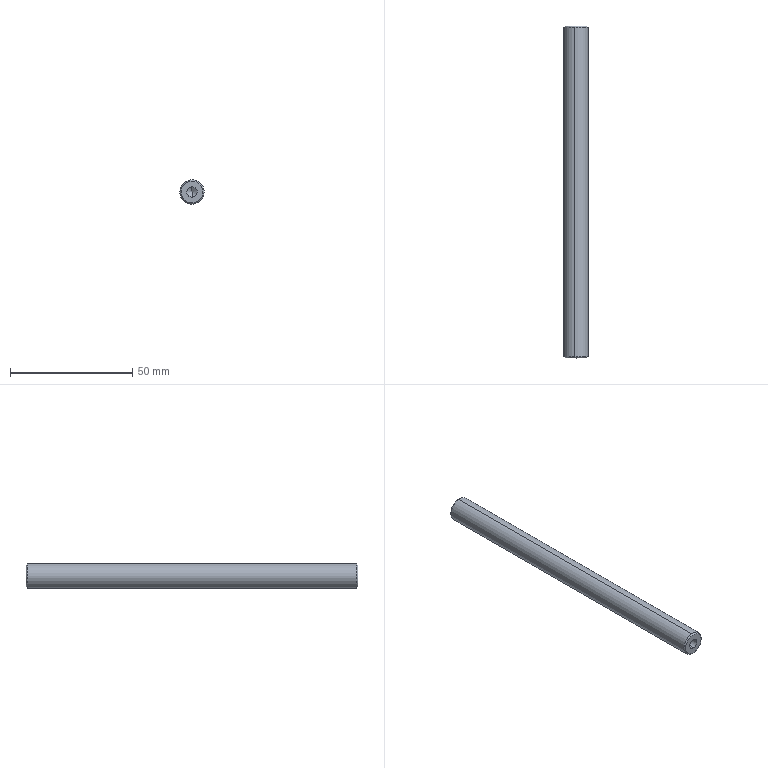Component | SolidWorks | BlankingGuidePost-136-1 | 1 solid | 16 faces | box 10 x 136 x 10 mm | volume 10319 mm3 | cone 8 | cylinder 6 | plane 2 | commonest cylinder face diameters 4.2 x4 10 x2 | material 45
build123d program:
from build123d import *

# Parameters (mm, degrees)
SKETCH1_R           = 5
BOSS_EXTRUDE1_DEPTH = 68
CHAMFER1_SIZE       = 0.5


with BuildPart() as part:
    # Sketch1 → Boss-Extrude1 (new, symmetric)
    with BuildSketch(Plane.XY):
        Circle(SKETCH1_R)
    extrude(amount=BOSS_EXTRUDE1_DEPTH, both=True)

    # Sketch4 → M5 Tapped Hole1 (revolve, cut)
    with BuildSketch(Plane(origin=(0, 0, 68), x_dir=(0, -1, 0), z_dir=(1, 0, 0))):
        Polygon((0, 0), (0, 13.662), (2.1, 12.4), (2.1, 0), align=None)
    m5_tapped_hole1 = revolve(axis=Axis((0, 0, 74.35), (0, 0, -1)), mode=Mode.SUBTRACT)

    # Mirror1: M5 Tapped Hole1 across plane
    add(m5_tapped_hole1.mirror(Plane.XY), mode=Mode.SUBTRACT)

    # Chamfer1
    chamfer1_edges = [part.edges().sort_by_distance(p)[0] for p in [
        (-5, 0, -68),
        (-5, 0, 68),
    ]]
    chamfer(chamfer1_edges, length=CHAMFER1_SIZE)


solid = part.part

# Placed as in the assembly
solid = solid.moved(Location((0, -25, -30), (90, 0, 0)))
STEP:
#1=CARTESIAN_POINT('',(-0.01499,-3.661,-1.005));
#2=VERTEX_POINT('',#1);
#3=CARTESIAN_POINT('',(0.01499,-3.661,-1.358));
#4=VERTEX_POINT('',#3);
#5=CARTESIAN_POINT('',(-0.,-3.661,-1.181));
#6=DIRECTION('',(0.,-1.,-0.));
#7=DIRECTION('',(-0.08459,0.,0.9964));
#8=AXIS2_PLACEMENT_3D('',#5,#6,#7);
#9=CIRCLE('',#8,0.1772);
#10=EDGE_CURVE('',#2,#4,#9,.T.);
#11=ORIENTED_EDGE('',*,*,#10,.F.);
#12=CARTESIAN_POINT('',(-0.01665,-3.642,-0.985));
#13=VERTEX_POINT('',#12);
#14=CARTESIAN_POINT('',(-0.01499,-3.661,-1.005));
#15=DIRECTION('',(-0.05981,0.7071,0.7046));
#16=VECTOR('',#15,39.37);
#17=LINE('',#14,#16);
#18=EDGE_CURVE('',#2,#13,#17,.T.);
#19=ORIENTED_EDGE('',*,*,#18,.T.);
#20=CARTESIAN_POINT('',(0.01665,-3.642,-1.377));
#21=VERTEX_POINT('',#20);
#22=CARTESIAN_POINT('',(-0.,-3.642,-1.181));
#23=DIRECTION('',(-0.,1.,0.));
#24=DIRECTION('',(-0.08459,0.,0.9964));
#25=AXIS2_PLACEMENT_3D('',#22,#23,#24);
#26=CIRCLE('',#25,0.1969);
#27=EDGE_CURVE('',#21,#13,#26,.T.);
#28=ORIENTED_EDGE('',*,*,#27,.F.);
#29=CARTESIAN_POINT('',(0.01499,-3.661,-1.358));
#30=DIRECTION('',(0.05981,0.7071,-0.7046));
#31=VECTOR('',#30,39.37);
#32=LINE('',#29,#31);
#33=EDGE_CURVE('',#4,#21,#32,.T.);
#34=ORIENTED_EDGE('',*,*,#33,.F.);
#35=EDGE_LOOP('',(#11,#19,#28,#34));
#36=FACE_OUTER_BOUND('',#35,.T.);
#37=CARTESIAN_POINT('',(-0.,-3.661,-1.181));
#38=DIRECTION('',(-0.,1.,0.));
#39=DIRECTION('',(0.08459,0.,-0.9964));
#40=AXIS2_PLACEMENT_3D('',#37,#38,#39);
#41=CONICAL_SURFACE('',#40,0.1772,0.7854);
#42=ADVANCED_FACE('',(#36),#41,.T.);
#43=CARTESIAN_POINT('',(0.01499,1.693,-1.358));
#44=VERTEX_POINT('',#43);
#45=CARTESIAN_POINT('',(-0.01499,1.693,-1.005));
#46=VERTEX_POINT('',#45);
#47=CARTESIAN_POINT('',(-0.,1.693,-1.181));
#48=DIRECTION('',(-0.,1.,0.));
#49=DIRECTION('',(-0.08459,0.,0.9964));
#50=AXIS2_PLACEMENT_3D('',#47,#48,#49);
#51=CIRCLE('',#50,0.1772);
#52=EDGE_CURVE('',#44,#46,#51,.T.);
#53=ORIENTED_EDGE('',*,*,#52,.F.);
#54=CARTESIAN_POINT('',(0.01665,1.673,-1.377));
#55=VERTEX_POINT('',#54);
#56=CARTESIAN_POINT('',(0.01665,1.673,-1.377));
#57=DIRECTION('',(0.05981,-0.7071,-0.7046));
#58=VECTOR('',#57,39.37);
#59=LINE('',#56,#58);
#60=EDGE_CURVE('',#44,#55,#59,.T.);
#61=ORIENTED_EDGE('',*,*,#60,.T.);
#62=CARTESIAN_POINT('',(-0.01665,1.673,-0.985));
#63=VERTEX_POINT('',#62);
#64=CARTESIAN_POINT('',(-0.,1.673,-1.181));
#65=DIRECTION('',(0.,-1.,-0.));
#66=DIRECTION('',(-0.08459,0.,0.9964));
#67=AXIS2_PLACEMENT_3D('',#64,#65,#66);
#68=CIRCLE('',#67,0.1969);
#69=EDGE_CURVE('',#63,#55,#68,.T.);
#70=ORIENTED_EDGE('',*,*,#69,.F.);
#71=CARTESIAN_POINT('',(-0.01665,1.673,-0.985));
#72=DIRECTION('',(-0.05981,-0.7071,0.7046));
#73=VECTOR('',#72,39.37);
#74=LINE('',#71,#73);
#75=EDGE_CURVE('',#46,#63,#74,.T.);
#76=ORIENTED_EDGE('',*,*,#75,.F.);
#77=EDGE_LOOP('',(#53,#61,#70,#76));
#78=FACE_OUTER_BOUND('',#77,.T.);
#79=CARTESIAN_POINT('',(-0.,1.673,-1.181));
#80=DIRECTION('',(0.,-1.,-0.));
#81=DIRECTION('',(-0.08459,0.,0.9964));
#82=AXIS2_PLACEMENT_3D('',#79,#80,#81);
#83=CONICAL_SURFACE('',#82,0.1969,0.7854);
#84=ADVANCED_FACE('',(#78),#83,.T.);
#85=CARTESIAN_POINT('',(-0.006994,1.205,-1.099));
#86=VERTEX_POINT('',#85);
#87=CARTESIAN_POINT('',(0.006994,1.205,-1.263));
#88=VERTEX_POINT('',#87);
#89=CARTESIAN_POINT('',(-0.,1.205,-1.181));
#90=DIRECTION('',(-0.,1.,0.));
#91=DIRECTION('',(0.08459,0.,-0.9964));
#92=AXIS2_PLACEMENT_3D('',#89,#90,#91);
#93=CIRCLE('',#92,0.08268);
#94=EDGE_CURVE('',#86,#88,#93,.T.);
#95=ORIENTED_EDGE('',*,*,#94,.F.);
#96=CARTESIAN_POINT('',(-0.006994,1.693,-1.099));
#97=VERTEX_POINT('',#96);
#98=CARTESIAN_POINT('',(-0.006994,1.693,-1.099));
#99=DIRECTION('',(-0.,1.,0.));
#100=VECTOR('',#99,39.37);
#101=LINE('',#98,#100);
#102=EDGE_CURVE('',#86,#97,#101,.T.);
#103=ORIENTED_EDGE('',*,*,#102,.T.);
#104=CARTESIAN_POINT('',(0.006994,1.693,-1.263));
#105=VERTEX_POINT('',#104);
#106=CARTESIAN_POINT('',(-0.,1.693,-1.181));
#107=DIRECTION('',(-0.,1.,0.));
#108=DIRECTION('',(0.08459,0.,-0.9964));
#109=AXIS2_PLACEMENT_3D('',#106,#107,#108);
#110=CIRCLE('',#109,0.08268);
#111=EDGE_CURVE('',#97,#105,#110,.T.);
#112=ORIENTED_EDGE('',*,*,#111,.T.);
#113=CARTESIAN_POINT('',(0.006994,1.693,-1.263));
#114=DIRECTION('',(-0.,1.,0.));
#115=VECTOR('',#114,39.37);
#116=LINE('',#113,#115);
#117=EDGE_CURVE('',#88,#105,#116,.T.);
#118=ORIENTED_EDGE('',*,*,#117,.F.);
#119=EDGE_LOOP('',(#95,#103,#112,#118));
#120=FACE_OUTER_BOUND('',#119,.T.);
#121=CARTESIAN_POINT('',(-0.,1.693,-1.181));
#122=DIRECTION('',(-0.,1.,0.));
#123=DIRECTION('',(0.08459,0.,-0.9964));
#124=AXIS2_PLACEMENT_3D('',#121,#122,#123);
#125=CYLINDRICAL_SURFACE('',#124,0.08268);
#126=ADVANCED_FACE('',(#120),#125,.F.);
#127=CARTESIAN_POINT('',(-0.,1.155,-1.181));
#128=VERTEX_POINT('',#127);
#129=CARTESIAN_POINT('',(0.006994,1.205,-1.263));
#130=DIRECTION('',(0.07251,0.515,-0.8541));
#131=VECTOR('',#130,39.37);
#132=LINE('',#129,#131);
#133=EDGE_CURVE('',#128,#88,#132,.T.);
#134=ORIENTED_EDGE('',*,*,#133,.F.);
#135=CARTESIAN_POINT('',(-0.006994,1.205,-1.099));
#136=DIRECTION('',(-0.07251,0.515,0.8541));
#137=VECTOR('',#136,39.37);
#138=LINE('',#135,#137);
#139=EDGE_CURVE('',#128,#86,#138,.T.);
#140=ORIENTED_EDGE('',*,*,#139,.T.);
#141=ORIENTED_EDGE('',*,*,#94,.T.);
#142=EDGE_LOOP('',(#134,#140,#141));
#143=FACE_OUTER_BOUND('',#142,.T.);
#144=CARTESIAN_POINT('',(-0.,1.205,-1.181));
#145=DIRECTION('',(-0.,1.,0.));
#146=DIRECTION('',(0.08459,0.,-0.9964));
#147=AXIS2_PLACEMENT_3D('',#144,#145,#146);
#148=CONICAL_SURFACE('',#147,0.08268,1.03);
#149=ADVANCED_FACE('',(#143),#148,.F.);
#150=CARTESIAN_POINT('',(0.006994,-3.173,-1.263));
#151=VERTEX_POINT('',#150);
#152=CARTESIAN_POINT('',(-0.006994,-3.173,-1.099));
#153=VERTEX_POINT('',#152);
#154=CARTESIAN_POINT('',(-0.,-3.173,-1.181));
#155=DIRECTION('',(0.,-1.,-0.));
#156=DIRECTION('',(-0.08459,0.,0.9964));
#157=AXIS2_PLACEMENT_3D('',#154,#155,#156);
#158=CIRCLE('',#157,0.08268);
#159=EDGE_CURVE('',#151,#153,#158,.T.);
#160=ORIENTED_EDGE('',*,*,#159,.F.);
#161=CARTESIAN_POINT('',(0.006994,-3.661,-1.263));
#162=VERTEX_POINT('',#161);
#163=CARTESIAN_POINT('',(0.006994,-3.661,-1.263));
#164=DIRECTION('',(0.,-1.,-0.));
#165=VECTOR('',#164,39.37);
#166=LINE('',#163,#165);
#167=EDGE_CURVE('',#151,#162,#166,.T.);
#168=ORIENTED_EDGE('',*,*,#167,.T.);
#169=CARTESIAN_POINT('',(-0.006994,-3.661,-1.099));
#170=VERTEX_POINT('',#169);
#171=CARTESIAN_POINT('',(-0.,-3.661,-1.181));
#172=DIRECTION('',(0.,-1.,-0.));
#173=DIRECTION('',(-0.08459,0.,0.9964));
#174=AXIS2_PLACEMENT_3D('',#171,#172,#173);
#175=CIRCLE('',#174,0.08268);
#176=EDGE_CURVE('',#162,#170,#175,.T.);
#177=ORIENTED_EDGE('',*,*,#176,.T.);
#178=CARTESIAN_POINT('',(-0.006994,-3.661,-1.099));
#179=DIRECTION('',(0.,-1.,-0.));
#180=VECTOR('',#179,39.37);
#181=LINE('',#178,#180);
#182=EDGE_CURVE('',#153,#170,#181,.T.);
#183=ORIENTED_EDGE('',*,*,#182,.F.);
#184=EDGE_LOOP('',(#160,#168,#177,#183));
#185=FACE_OUTER_BOUND('',#184,.T.);
#186=CARTESIAN_POINT('',(-0.,-3.661,-1.181));
#187=DIRECTION('',(0.,-1.,-0.));
#188=DIRECTION('',(-0.08459,0.,0.9964));
#189=AXIS2_PLACEMENT_3D('',#186,#187,#188);
#190=CYLINDRICAL_SURFACE('',#189,0.08268);
#191=ADVANCED_FACE('',(#185),#190,.F.);
#192=CARTESIAN_POINT('',(-0.,-3.124,-1.181));
#193=VERTEX_POINT('',#192);
#194=CARTESIAN_POINT('',(-0.006994,-3.173,-1.099));
#195=DIRECTION('',(-0.07251,-0.515,0.8541));
#196=VECTOR('',#195,39.37);
#197=LINE('',#194,#196);
#198=EDGE_CURVE('',#193,#153,#197,.T.);
#199=ORIENTED_EDGE('',*,*,#198,.F.);
#200=CARTESIAN_POINT('',(0.006994,-3.173,-1.263));
#201=DIRECTION('',(0.07251,-0.515,-0.8541));
#202=VECTOR('',#201,39.37);
#203=LINE('',#200,#202);
#204=EDGE_CURVE('',#193,#151,#203,.T.);
#205=ORIENTED_EDGE('',*,*,#204,.T.);
#206=ORIENTED_EDGE('',*,*,#159,.T.);
#207=EDGE_LOOP('',(#199,#205,#206));
#208=FACE_OUTER_BOUND('',#207,.T.);
#209=CARTESIAN_POINT('',(-0.,-3.173,-1.181));
#210=DIRECTION('',(0.,-1.,-0.));
#211=DIRECTION('',(-0.08459,0.,0.9964));
#212=AXIS2_PLACEMENT_3D('',#209,#210,#211);
#213=CONICAL_SURFACE('',#212,0.08268,1.03);
#214=ADVANCED_FACE('',(#208),#213,.F.);
#215=ORIENTED_EDGE('',*,*,#27,.T.);
#216=CARTESIAN_POINT('',(-0.01665,-3.661,-0.985));
#217=DIRECTION('',(-0.,1.,0.));
#218=VECTOR('',#217,39.37);
#219=LINE('',#216,#218);
#220=EDGE_CURVE('',#13,#63,#219,.T.);
#221=ORIENTED_EDGE('',*,*,#220,.T.);
#222=ORIENTED_EDGE('',*,*,#69,.T.);
#223=CARTESIAN_POINT('',(0.01665,-3.661,-1.377));
#224=DIRECTION('',(-0.,1.,0.));
#225=VECTOR('',#224,39.37);
#226=LINE('',#223,#225);
#227=EDGE_CURVE('',#21,#55,#226,.T.);
#228=ORIENTED_EDGE('',*,*,#227,.F.);
#229=EDGE_LOOP('',(#215,#221,#222,#228));
#230=FACE_OUTER_BOUND('',#229,.T.);
#231=CARTESIAN_POINT('',(-0.,-3.661,-1.181));
#232=DIRECTION('',(-0.,1.,0.));
#233=DIRECTION('',(0.08459,0.,-0.9964));
#234=AXIS2_PLACEMENT_3D('',#231,#232,#233);
#235=CYLINDRICAL_SURFACE('',#234,0.1969);
#236=ADVANCED_FACE('',(#230),#235,.T.);
#237=ORIENTED_EDGE('',*,*,#220,.F.);
#238=CARTESIAN_POINT('',(-0.,-3.642,-1.181));
#239=DIRECTION('',(-0.,1.,0.));
#240=DIRECTION('',(-0.08459,0.,0.9964));
#241=AXIS2_PLACEMENT_3D('',#238,#239,#240);
#242=CIRCLE('',#241,0.1969);
#243=EDGE_CURVE('',#13,#21,#242,.T.);
#244=ORIENTED_EDGE('',*,*,#243,.T.);
#245=ORIENTED_EDGE('',*,*,#227,.T.);
#246=CARTESIAN_POINT('',(-0.,1.673,-1.181));
#247=DIRECTION('',(0.,-1.,-0.));
#248=DIRECTION('',(-0.08459,0.,0.9964));
#249=AXIS2_PLACEMENT_3D('',#246,#247,#248);
#250=CIRCLE('',#249,0.1969);
#251=EDGE_CURVE('',#55,#63,#250,.T.);
#252=ORIENTED_EDGE('',*,*,#251,.T.);
#253=EDGE_LOOP('',(#237,#244,#245,#252));
#254=FACE_OUTER_BOUND('',#253,.T.);
#255=CARTESIAN_POINT('',(-0.,-3.661,-1.181));
#256=DIRECTION('',(-0.,1.,0.));
#257=DIRECTION('',(0.08459,0.,-0.9964));
#258=AXIS2_PLACEMENT_3D('',#255,#256,#257);
#259=CYLINDRICAL_SURFACE('',#258,0.1969);
#260=ADVANCED_FACE('',(#254),#259,.T.);
#261=CARTESIAN_POINT('',(-0.,-3.661,-1.181));
#262=DIRECTION('',(0.,-1.,-0.));
#263=DIRECTION('',(-0.08459,0.,0.9964));
#264=AXIS2_PLACEMENT_3D('',#261,#262,#263);
#265=CIRCLE('',#264,0.1772);
#266=EDGE_CURVE('',#4,#2,#265,.T.);
#267=ORIENTED_EDGE('',*,*,#266,.T.);
#268=ORIENTED_EDGE('',*,*,#10,.T.);
#269=EDGE_LOOP('',(#267,#268));
#270=FACE_OUTER_BOUND('',#269,.T.);
#271=CARTESIAN_POINT('',(-0.,-3.661,-1.181));
#272=DIRECTION('',(0.,-1.,-0.));
#273=DIRECTION('',(-0.08459,0.,0.9964));
#274=AXIS2_PLACEMENT_3D('',#271,#272,#273);
#275=CIRCLE('',#274,0.08268);
#276=EDGE_CURVE('',#170,#162,#275,.T.);
#277=ORIENTED_EDGE('',*,*,#276,.F.);
#278=ORIENTED_EDGE('',*,*,#176,.F.);
#279=EDGE_LOOP('',(#277,#278));
#280=FACE_BOUND('',#279,.T.);
#281=CARTESIAN_POINT('',(-0.,-3.661,-1.181));
#282=DIRECTION('',(0.,-1.,-0.));
#283=DIRECTION('',(-0.08459,-0.,0.9964));
#284=AXIS2_PLACEMENT_3D('',#281,#282,#283);
#285=PLANE('',#284);
#286=ADVANCED_FACE('',(#270,#280),#285,.T.);
#287=CARTESIAN_POINT('',(-0.,1.693,-1.181));
#288=DIRECTION('',(-0.,1.,0.));
#289=DIRECTION('',(-0.08459,0.,0.9964));
#290=AXIS2_PLACEMENT_3D('',#287,#288,#289);
#291=CIRCLE('',#290,0.1772);
#292=EDGE_CURVE('',#46,#44,#291,.T.);
#293=ORIENTED_EDGE('',*,*,#292,.T.);
#294=ORIENTED_EDGE('',*,*,#52,.T.);
#295=EDGE_LOOP('',(#293,#294));
#296=FACE_OUTER_BOUND('',#295,.T.);
#297=CARTESIAN_POINT('',(-0.,1.693,-1.181));
#298=DIRECTION('',(-0.,1.,0.));
#299=DIRECTION('',(0.08459,0.,-0.9964));
#300=AXIS2_PLACEMENT_3D('',#297,#298,#299);
#301=CIRCLE('',#300,0.08268);
#302=EDGE_CURVE('',#105,#97,#301,.T.);
#303=ORIENTED_EDGE('',*,*,#302,.F.);
#304=ORIENTED_EDGE('',*,*,#111,.F.);
#305=EDGE_LOOP('',(#303,#304));
#306=FACE_BOUND('',#305,.T.);
#307=CARTESIAN_POINT('',(-0.,1.693,-1.181));
#308=DIRECTION('',(0.,-1.,-0.));
#309=DIRECTION('',(-0.08459,-0.,0.9964));
#310=AXIS2_PLACEMENT_3D('',#307,#308,#309);
#311=PLANE('',#310);
#312=ADVANCED_FACE('',(#296,#306),#311,.F.);
#313=ORIENTED_EDGE('',*,*,#204,.F.);
#314=ORIENTED_EDGE('',*,*,#198,.T.);
#315=CARTESIAN_POINT('',(-0.,-3.173,-1.181));
#316=DIRECTION('',(0.,-1.,-0.));
#317=DIRECTION('',(-0.08459,0.,0.9964));
#318=AXIS2_PLACEMENT_3D('',#315,#316,#317);
#319=CIRCLE('',#318,0.08268);
#320=EDGE_CURVE('',#153,#151,#319,.T.);
#321=ORIENTED_EDGE('',*,*,#320,.T.);
#322=EDGE_LOOP('',(#313,#314,#321));
#323=FACE_OUTER_BOUND('',#322,.T.);
#324=CARTESIAN_POINT('',(-0.,-3.173,-1.181));
#325=DIRECTION('',(0.,-1.,-0.));
#326=DIRECTION('',(-0.08459,0.,0.9964));
#327=AXIS2_PLACEMENT_3D('',#324,#325,#326);
#328=CONICAL_SURFACE('',#327,0.08268,1.03);
#329=ADVANCED_FACE('',(#323),#328,.F.);
#330=ORIENTED_EDGE('',*,*,#167,.F.);
#331=ORIENTED_EDGE('',*,*,#320,.F.);
#332=ORIENTED_EDGE('',*,*,#182,.T.);
#333=ORIENTED_EDGE('',*,*,#276,.T.);
#334=EDGE_LOOP('',(#330,#331,#332,#333));
#335=FACE_OUTER_BOUND('',#334,.T.);
#336=CARTESIAN_POINT('',(-0.,-3.661,-1.181));
#337=DIRECTION('',(0.,-1.,-0.));
#338=DIRECTION('',(-0.08459,0.,0.9964));
#339=AXIS2_PLACEMENT_3D('',#336,#337,#338);
#340=CYLINDRICAL_SURFACE('',#339,0.08268);
#341=ADVANCED_FACE('',(#335),#340,.F.);
#342=ORIENTED_EDGE('',*,*,#139,.F.);
#343=ORIENTED_EDGE('',*,*,#133,.T.);
#344=CARTESIAN_POINT('',(-0.,1.205,-1.181));
#345=DIRECTION('',(-0.,1.,0.));
#346=DIRECTION('',(0.08459,0.,-0.9964));
#347=AXIS2_PLACEMENT_3D('',#344,#345,#346);
#348=CIRCLE('',#347,0.08268);
#349=EDGE_CURVE('',#88,#86,#348,.T.);
#350=ORIENTED_EDGE('',*,*,#349,.T.);
#351=EDGE_LOOP('',(#342,#343,#350));
#352=FACE_OUTER_BOUND('',#351,.T.);
#353=CARTESIAN_POINT('',(-0.,1.205,-1.181));
#354=DIRECTION('',(-0.,1.,0.));
#355=DIRECTION('',(0.08459,0.,-0.9964));
#356=AXIS2_PLACEMENT_3D('',#353,#354,#355);
#357=CONICAL_SURFACE('',#356,0.08268,1.03);
#358=ADVANCED_FACE('',(#352),#357,.F.);
#359=ORIENTED_EDGE('',*,*,#102,.F.);
#360=ORIENTED_EDGE('',*,*,#349,.F.);
#361=ORIENTED_EDGE('',*,*,#117,.T.);
#362=ORIENTED_EDGE('',*,*,#302,.T.);
#363=EDGE_LOOP('',(#359,#360,#361,#362));
#364=FACE_OUTER_BOUND('',#363,.T.);
#365=CARTESIAN_POINT('',(-0.,1.693,-1.181));
#366=DIRECTION('',(-0.,1.,0.));
#367=DIRECTION('',(0.08459,0.,-0.9964));
#368=AXIS2_PLACEMENT_3D('',#365,#366,#367);
#369=CYLINDRICAL_SURFACE('',#368,0.08268);
#370=ADVANCED_FACE('',(#364),#369,.F.);
#371=ORIENTED_EDGE('',*,*,#60,.F.);
#372=ORIENTED_EDGE('',*,*,#292,.F.);
#373=ORIENTED_EDGE('',*,*,#75,.T.);
#374=ORIENTED_EDGE('',*,*,#251,.F.);
#375=EDGE_LOOP('',(#371,#372,#373,#374));
#376=FACE_OUTER_BOUND('',#375,.T.);
#377=CARTESIAN_POINT('',(-0.,1.673,-1.181));
#378=DIRECTION('',(0.,-1.,-0.));
#379=DIRECTION('',(-0.08459,0.,0.9964));
#380=AXIS2_PLACEMENT_3D('',#377,#378,#379);
#381=CONICAL_SURFACE('',#380,0.1969,0.7854);
#382=ADVANCED_FACE('',(#376),#381,.T.);
#383=ORIENTED_EDGE('',*,*,#18,.F.);
#384=ORIENTED_EDGE('',*,*,#266,.F.);
#385=ORIENTED_EDGE('',*,*,#33,.T.);
#386=ORIENTED_EDGE('',*,*,#243,.F.);
#387=EDGE_LOOP('',(#383,#384,#385,#386));
#388=FACE_OUTER_BOUND('',#387,.T.);
#389=CARTESIAN_POINT('',(-0.,-3.661,-1.181));
#390=DIRECTION('',(-0.,1.,0.));
#391=DIRECTION('',(0.08459,0.,-0.9964));
#392=AXIS2_PLACEMENT_3D('',#389,#390,#391);
#393=CONICAL_SURFACE('',#392,0.1772,0.7854);
#394=ADVANCED_FACE('',(#388),#393,.T.);
#395=CLOSED_SHELL('',(#42,#84,#126,#149,#191,#214,#236,#260,#286,#312,#329,#341,#358,#370,#382,#394));
#396=MANIFOLD_SOLID_BREP('',#395);
#397=CARTESIAN_POINT('',(0.,0.,0.));
#398=DIRECTION('',(0.,0.,1.));
#399=DIRECTION('',(1.,0.,0.));
#400=AXIS2_PLACEMENT_3D('',#397,#398,#399);
#401=(LENGTH_UNIT()NAMED_UNIT(*)SI_UNIT($,.METRE.));
#402=LENGTH_MEASURE_WITH_UNIT(LENGTH_MEASURE(0.0254),#401);
#403=DIMENSIONAL_EXPONENTS(1.,0.,0.,0.,0.,0.,0.);
#404=(CONVERSION_BASED_UNIT('',#402)LENGTH_UNIT()NAMED_UNIT(#403));
#405=UNCERTAINTY_MEASURE_WITH_UNIT(LENGTH_MEASURE(0.00001),#404,'','');
#406=(NAMED_UNIT(*)PLANE_ANGLE_UNIT()SI_UNIT($,.RADIAN.));
#407=(NAMED_UNIT(*)SI_UNIT($,.STERADIAN.)SOLID_ANGLE_UNIT());
#408=(GEOMETRIC_REPRESENTATION_CONTEXT(3)GLOBAL_UNCERTAINTY_ASSIGNED_CONTEXT((#405))GLOBAL_UNIT_ASSIGNED_CONTEXT((#404,#406,#407))REPRESENTATION_CONTEXT('',''));
#409=ADVANCED_BREP_SHAPE_REPRESENTATION('',(#396,#400),#408);
#410=COLOUR_RGB('',0.7922,0.8196,0.9333);
#411=FILL_AREA_STYLE_COLOUR('',#410);
#412=FILL_AREA_STYLE('',(#411));
#413=SURFACE_STYLE_FILL_AREA(#412);
#414=SURFACE_SIDE_STYLE('',(#413));
#415=SURFACE_STYLE_USAGE(.BOTH.,#414);
#416=PRESENTATION_STYLE_ASSIGNMENT((#415));
#417=STYLED_ITEM('',(#416),#396);
#418=PRESENTATION_LAYER_ASSIGNMENT('','',(#417));
#419=(LENGTH_UNIT()NAMED_UNIT(*)SI_UNIT($,.METRE.));
#420=LENGTH_MEASURE_WITH_UNIT(LENGTH_MEASURE(0.0254),#419);
#421=DIMENSIONAL_EXPONENTS(1.,0.,0.,0.,0.,0.,0.);
#422=(CONVERSION_BASED_UNIT('',#420)LENGTH_UNIT()NAMED_UNIT(#421));
#423=UNCERTAINTY_MEASURE_WITH_UNIT(LENGTH_MEASURE(0.00001),#422,'','');
#424=(NAMED_UNIT(*)PLANE_ANGLE_UNIT()SI_UNIT($,.RADIAN.));
#425=(NAMED_UNIT(*)SI_UNIT($,.STERADIAN.)SOLID_ANGLE_UNIT());
#426=(GEOMETRIC_REPRESENTATION_CONTEXT(3)GLOBAL_UNCERTAINTY_ASSIGNED_CONTEXT((#423))GLOBAL_UNIT_ASSIGNED_CONTEXT((#422,#424,#425))REPRESENTATION_CONTEXT('',''));
#427=MECHANICAL_DESIGN_GEOMETRIC_PRESENTATION_REPRESENTATION('',(#417),#426);